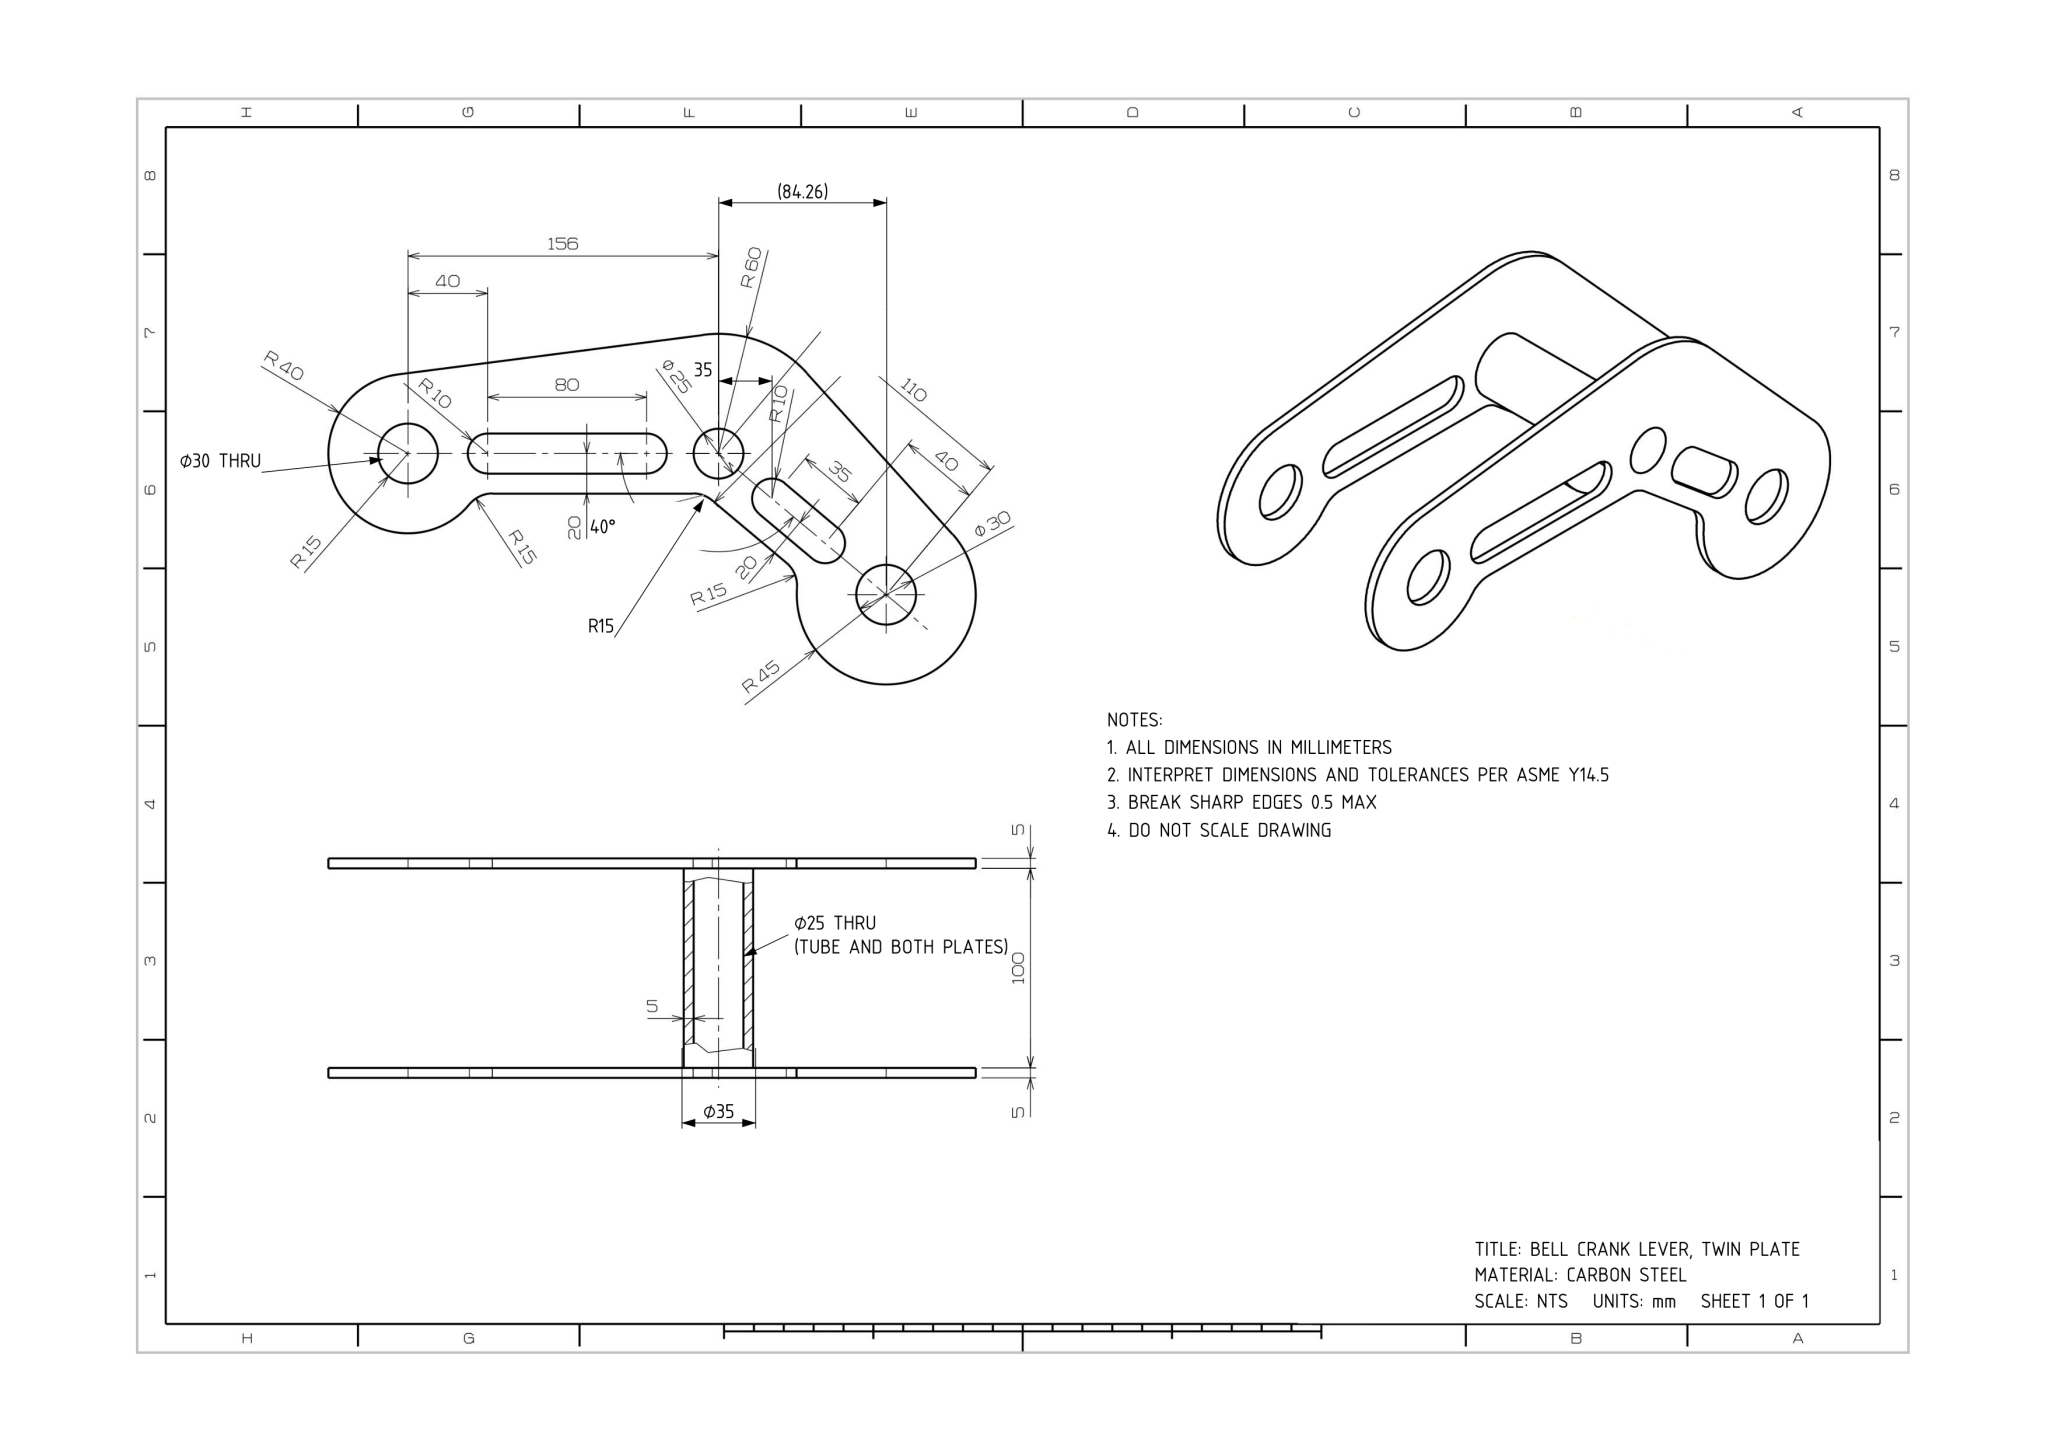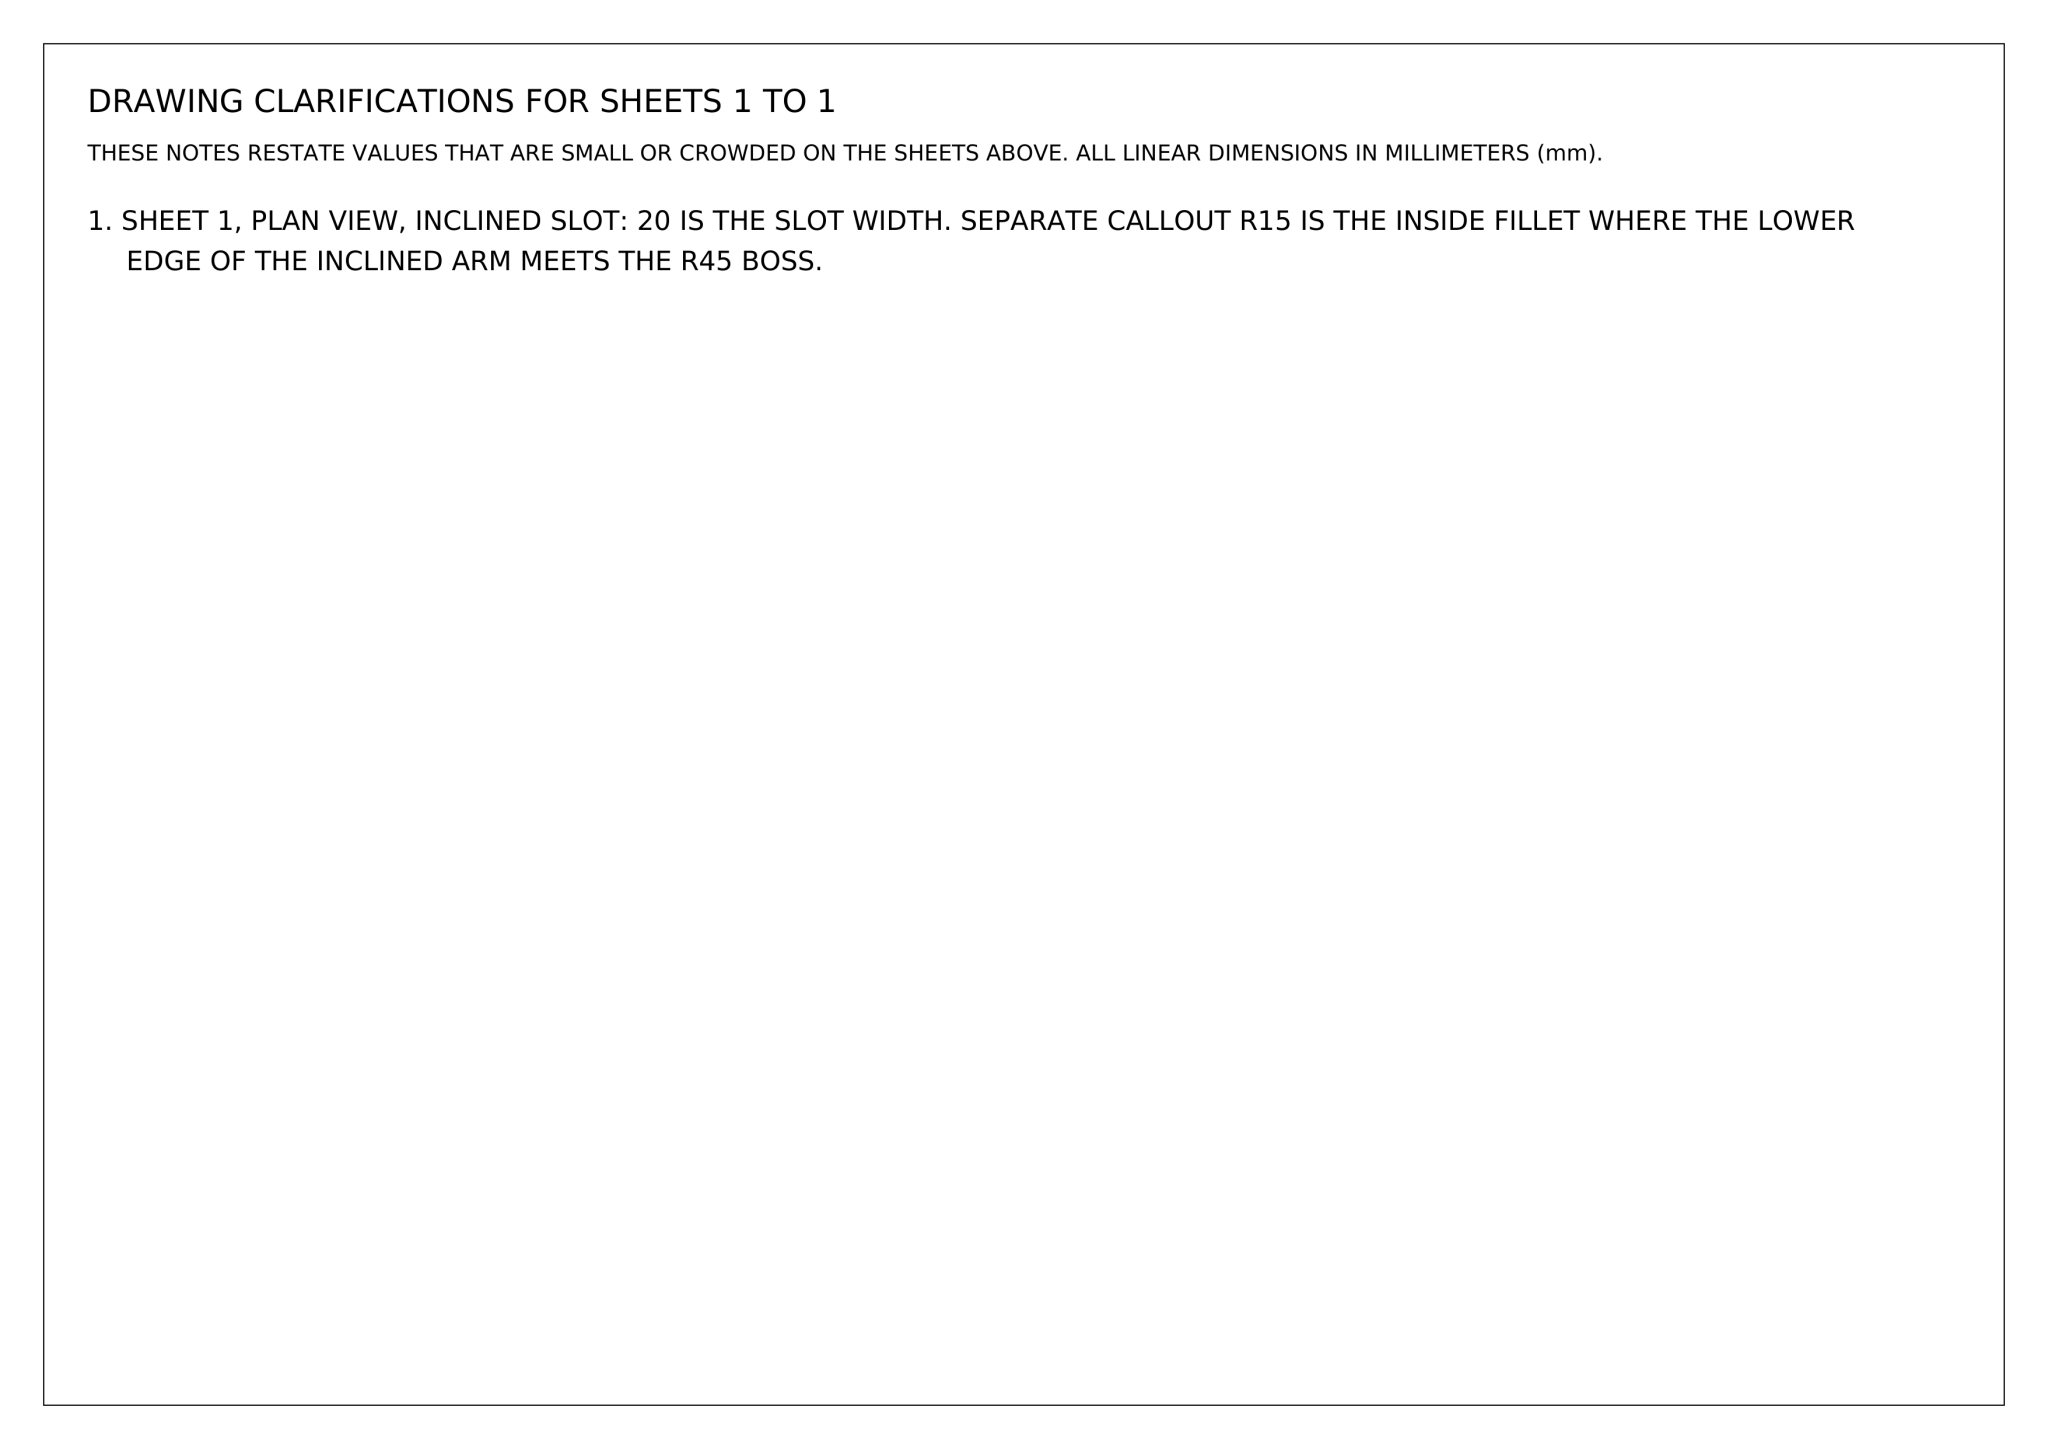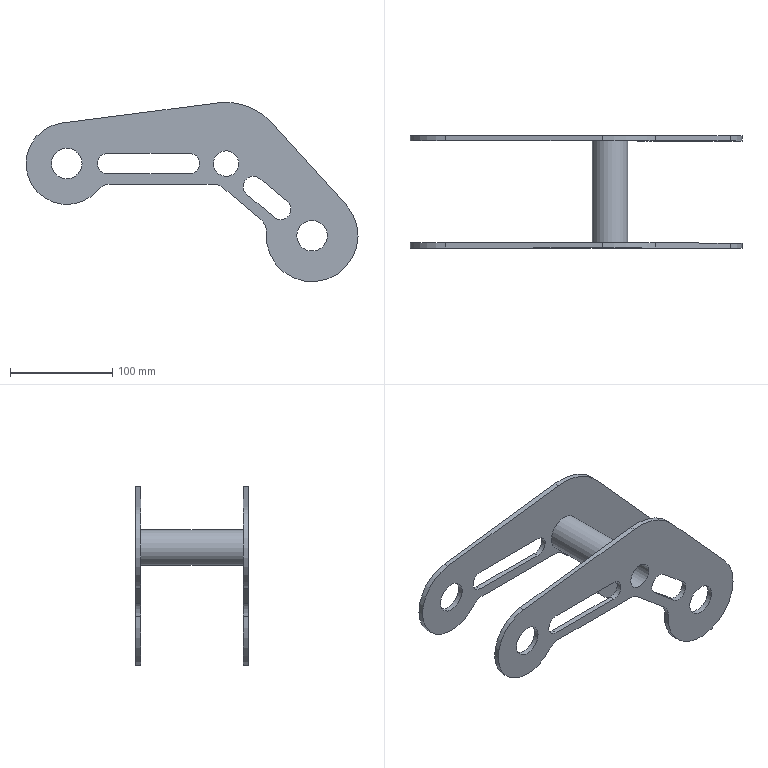Part | NX | mm | 1 solid | 46 faces | box 325.26 x 110 x 175.71 mm | volume 269320 mm3 | cylinder 26 | plane 20 | commonest cylinder face diameters 30 x10 20 x8 80 x2 90 x2 120 x2 35 x1 25 x1